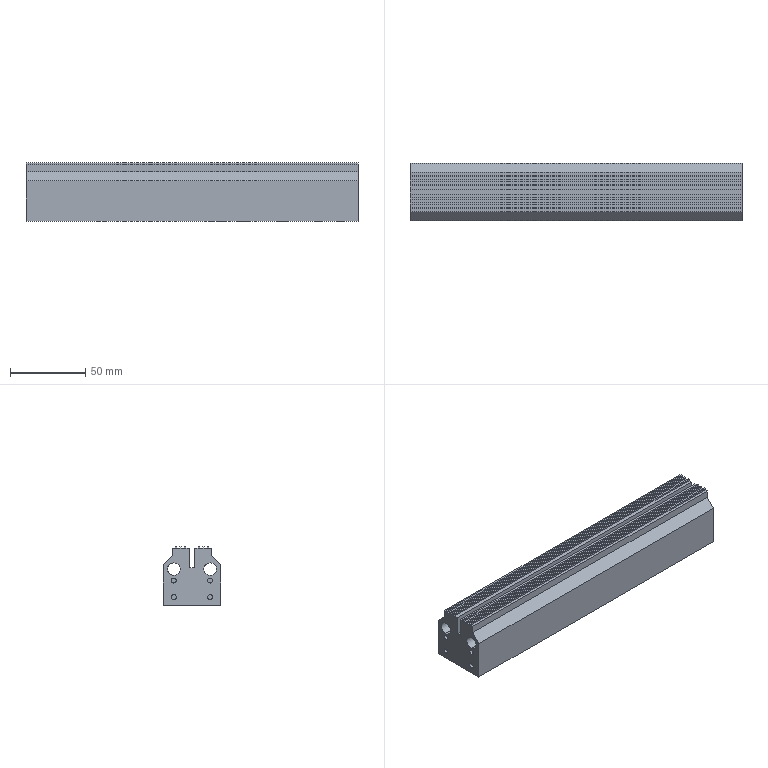CAM job | Mastercam | mm | 15 operations | part box 220 x 38 x 39
1. Contour (Ramp) | 4 - 6 平铣刀
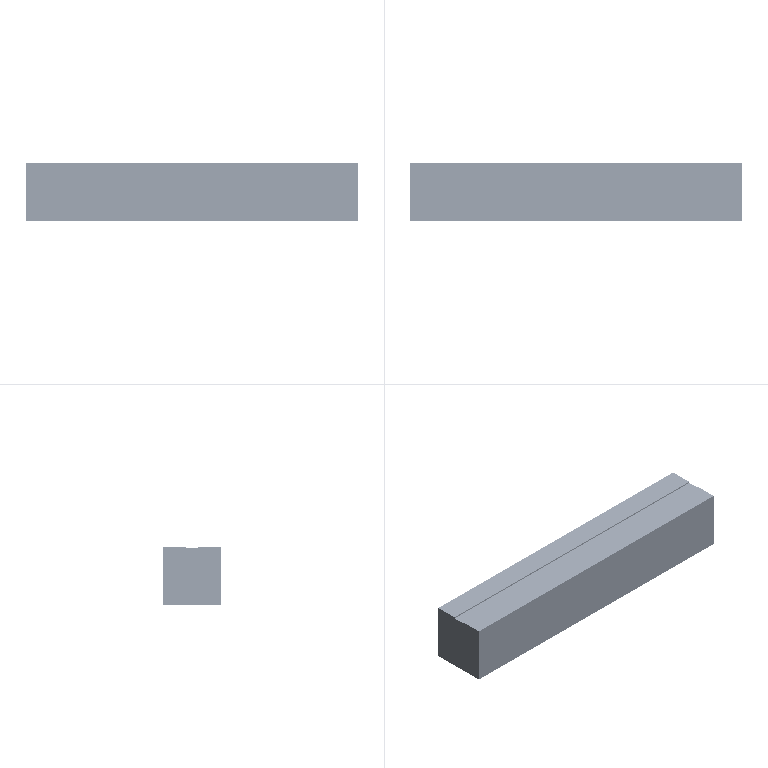2. Contour (Ramp) | 2 - 12 平铣刀
3. Surface Finish Flowline | 2 - 12 平铣刀
4. Contour (2D) | 5 - 6 平铣刀
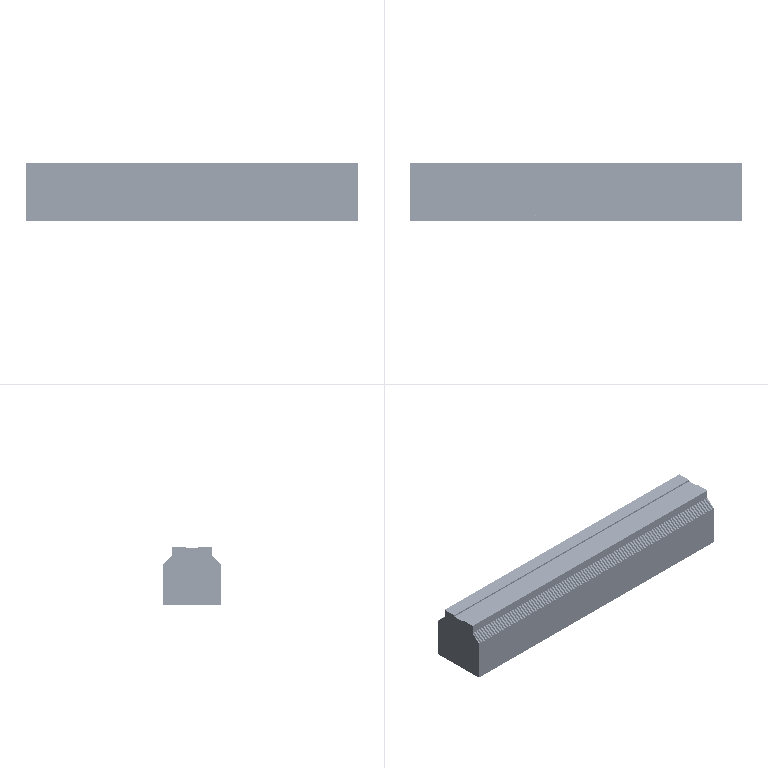5. Contour (2D) | 3 - 12 平铣刀
6. Contour (Ramp) | 15 - 3 平铣刀
7. Contour (Ramp) | 15 - 3 平铣刀
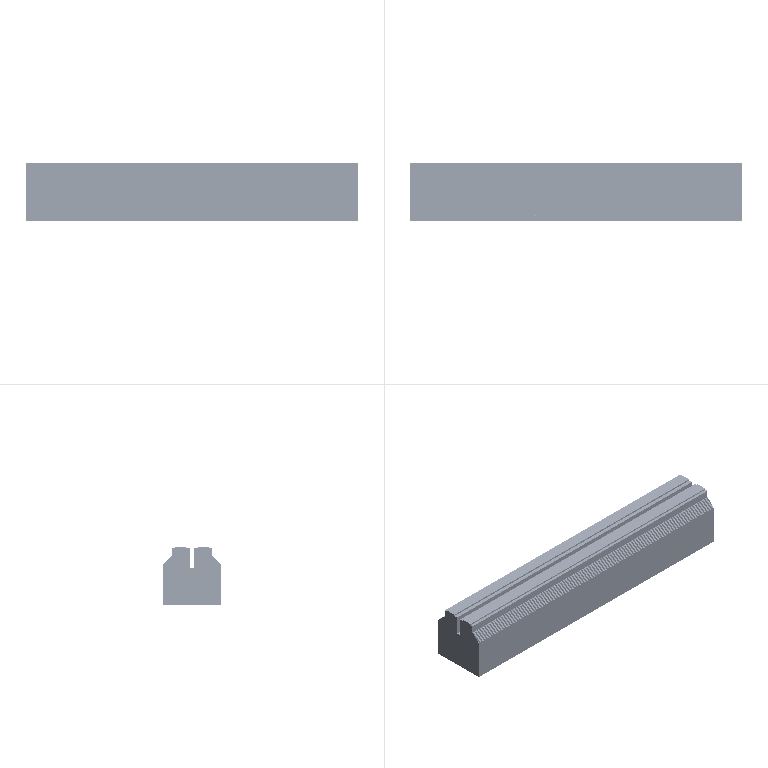8. Contour (2D) | 16 - 3 平铣刀
9. Contour (2D) | 16 - 3 平铣刀
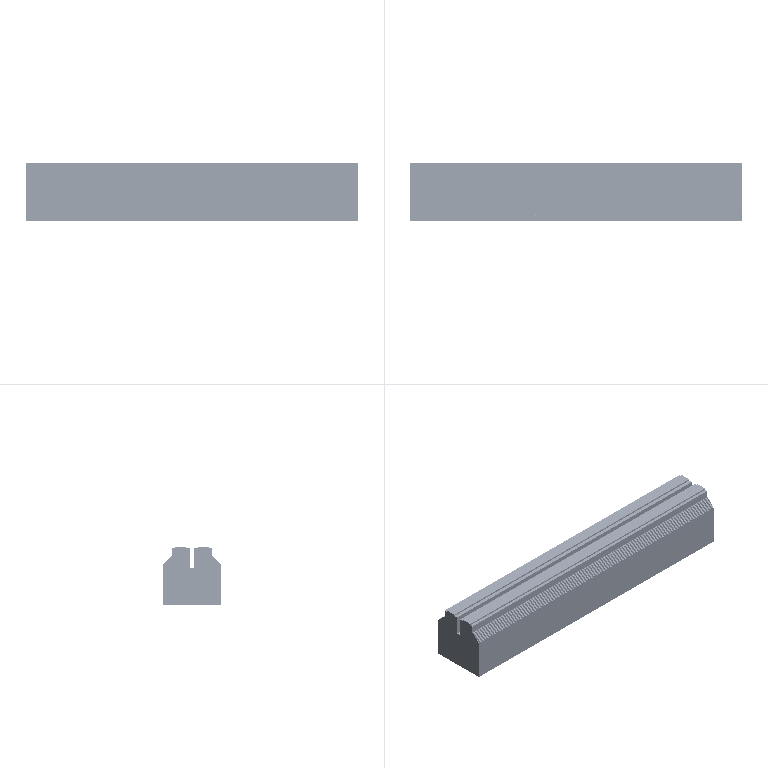10. Surface Finish Flowline | 7 - 17 圆鼻铣刀
11. Contour (Ramp) | 17 - 2 平铣刀
12. Contour (2D) | 18 - 2 平铣刀
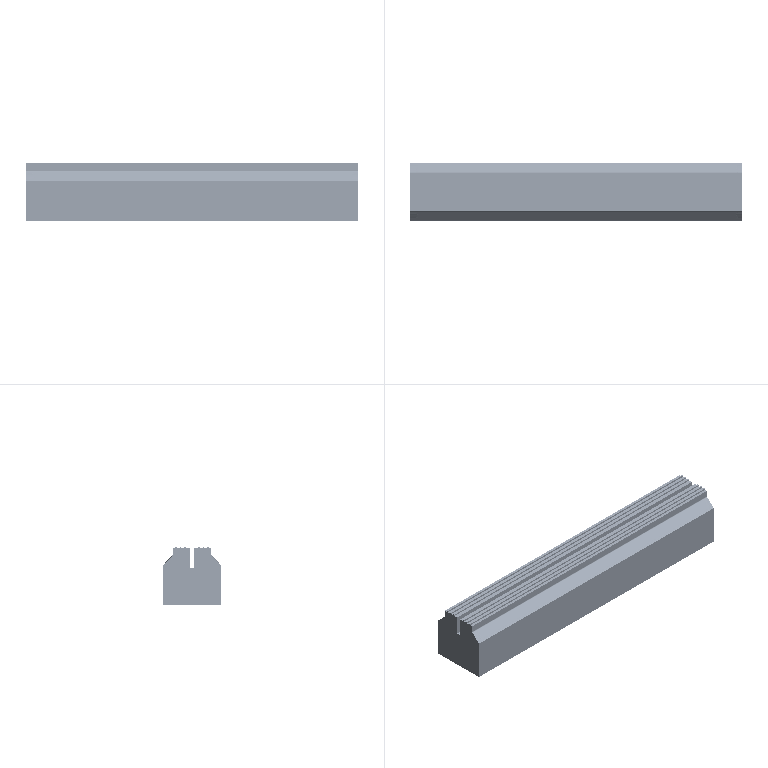13. Drill/Counterbore | 6 - 6 倒角刀
14. Peck Drill | 11 - 3.3 钻头
15. Chamfer Drill | 6 - 6 倒角刀